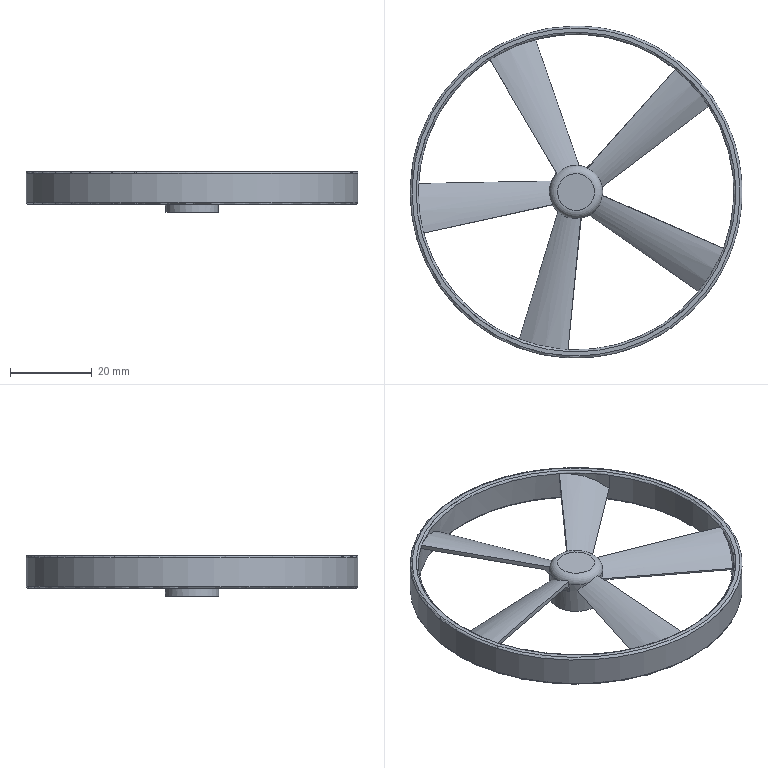Component | NX | FAN_BLADE | 1 solid | 43 faces | volume 6696 mm3 | spline 25 | plane 9 | torus 5 | cylinder 4 | commonest cylinder face diameters 77 x2 13 x1 81 x1